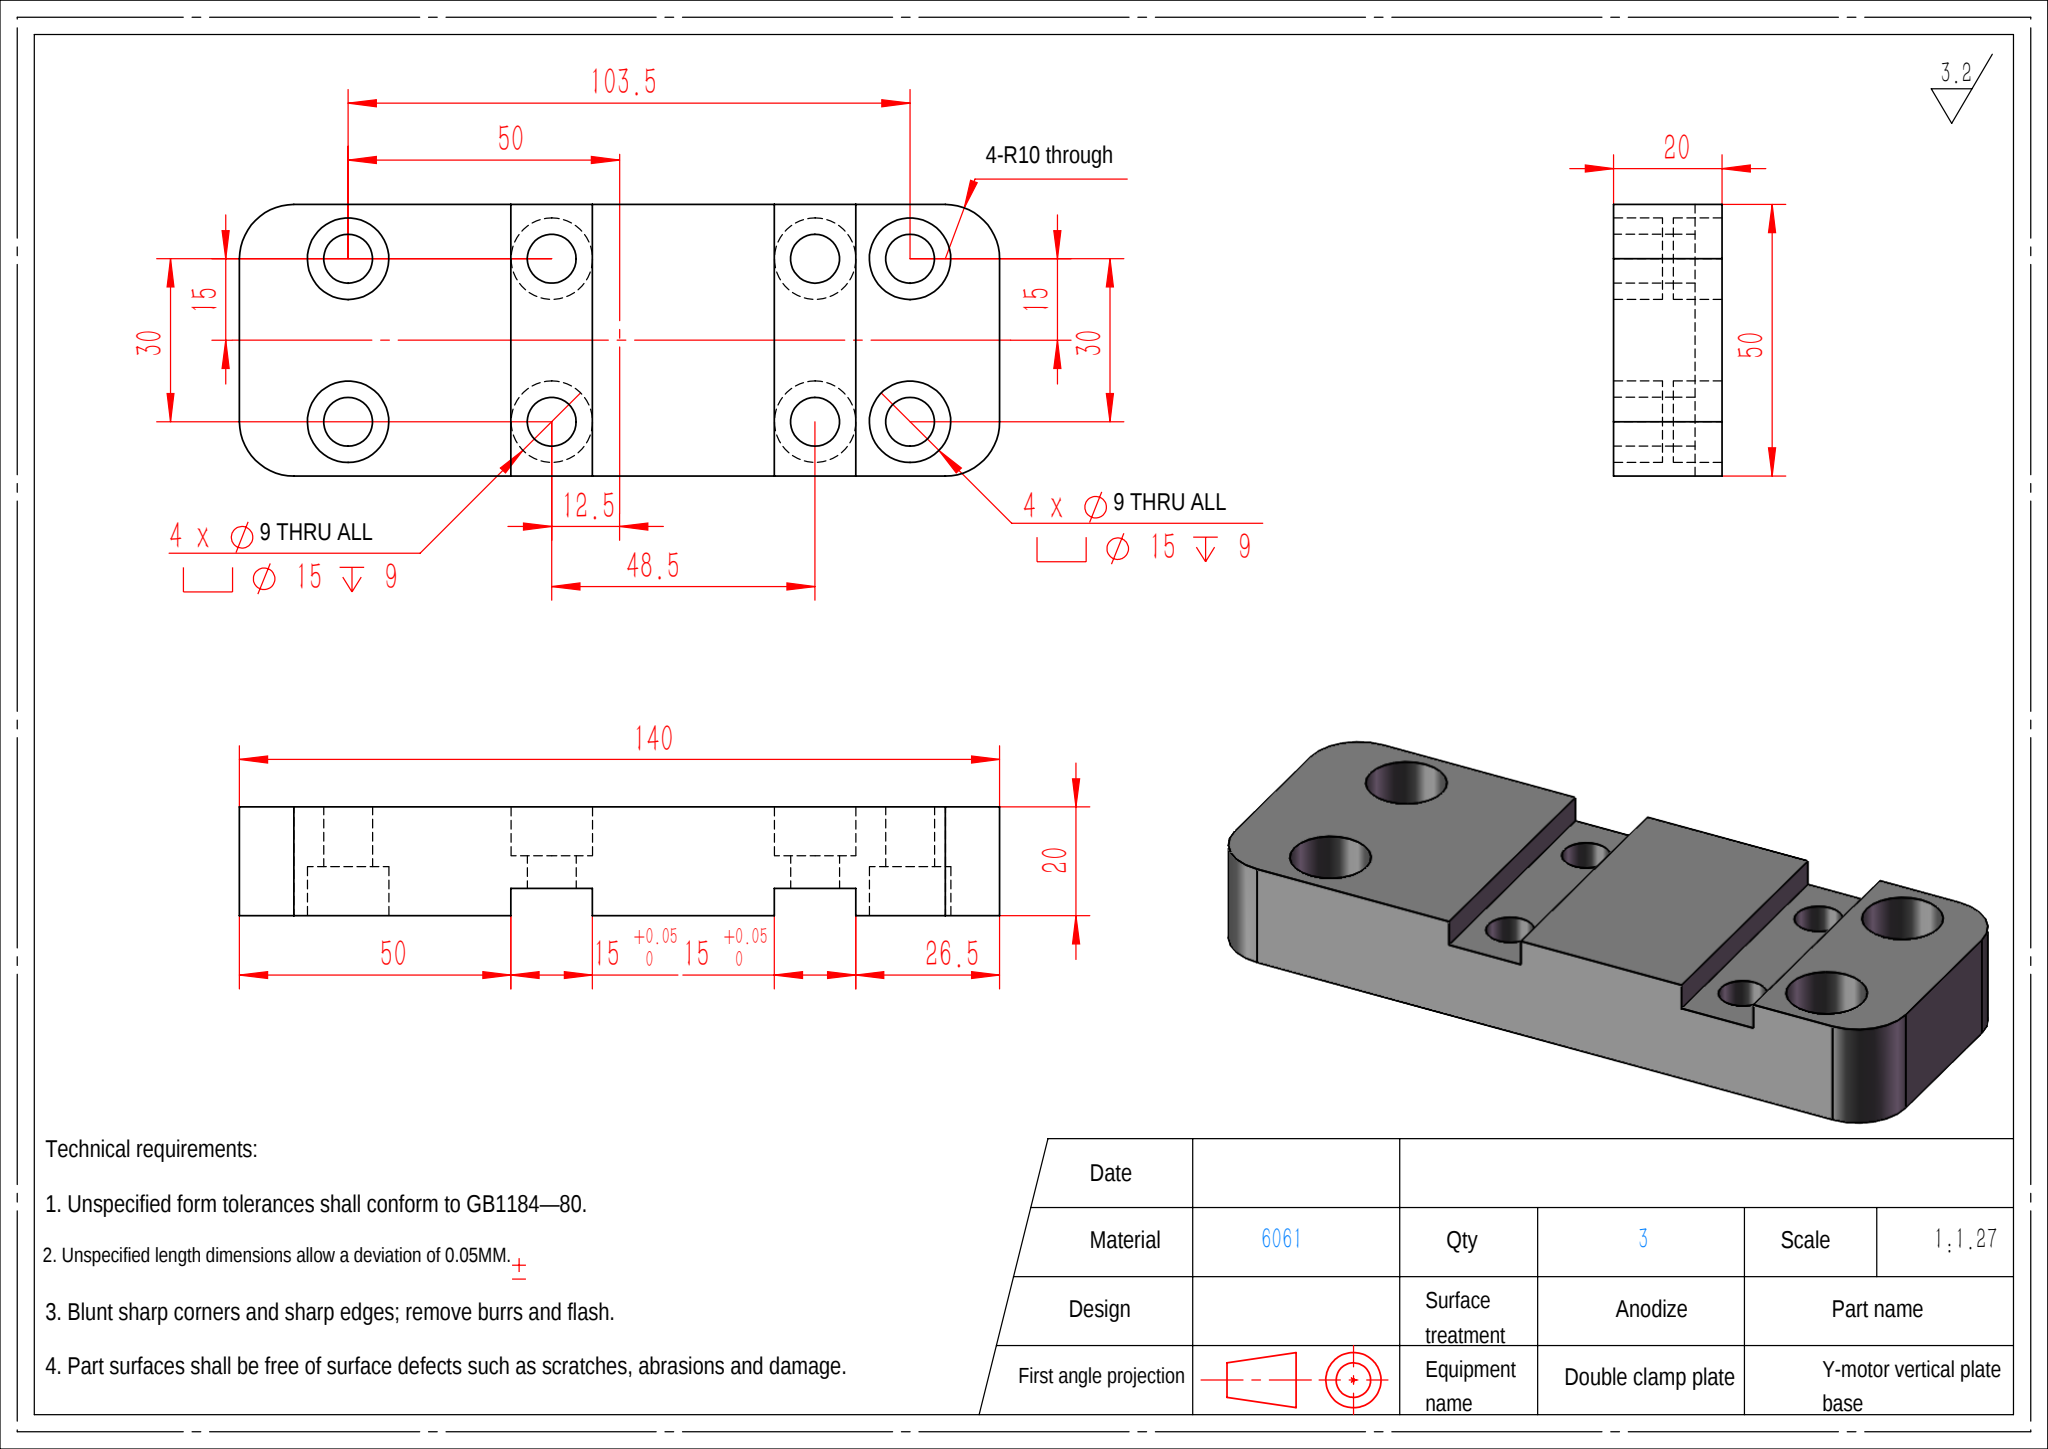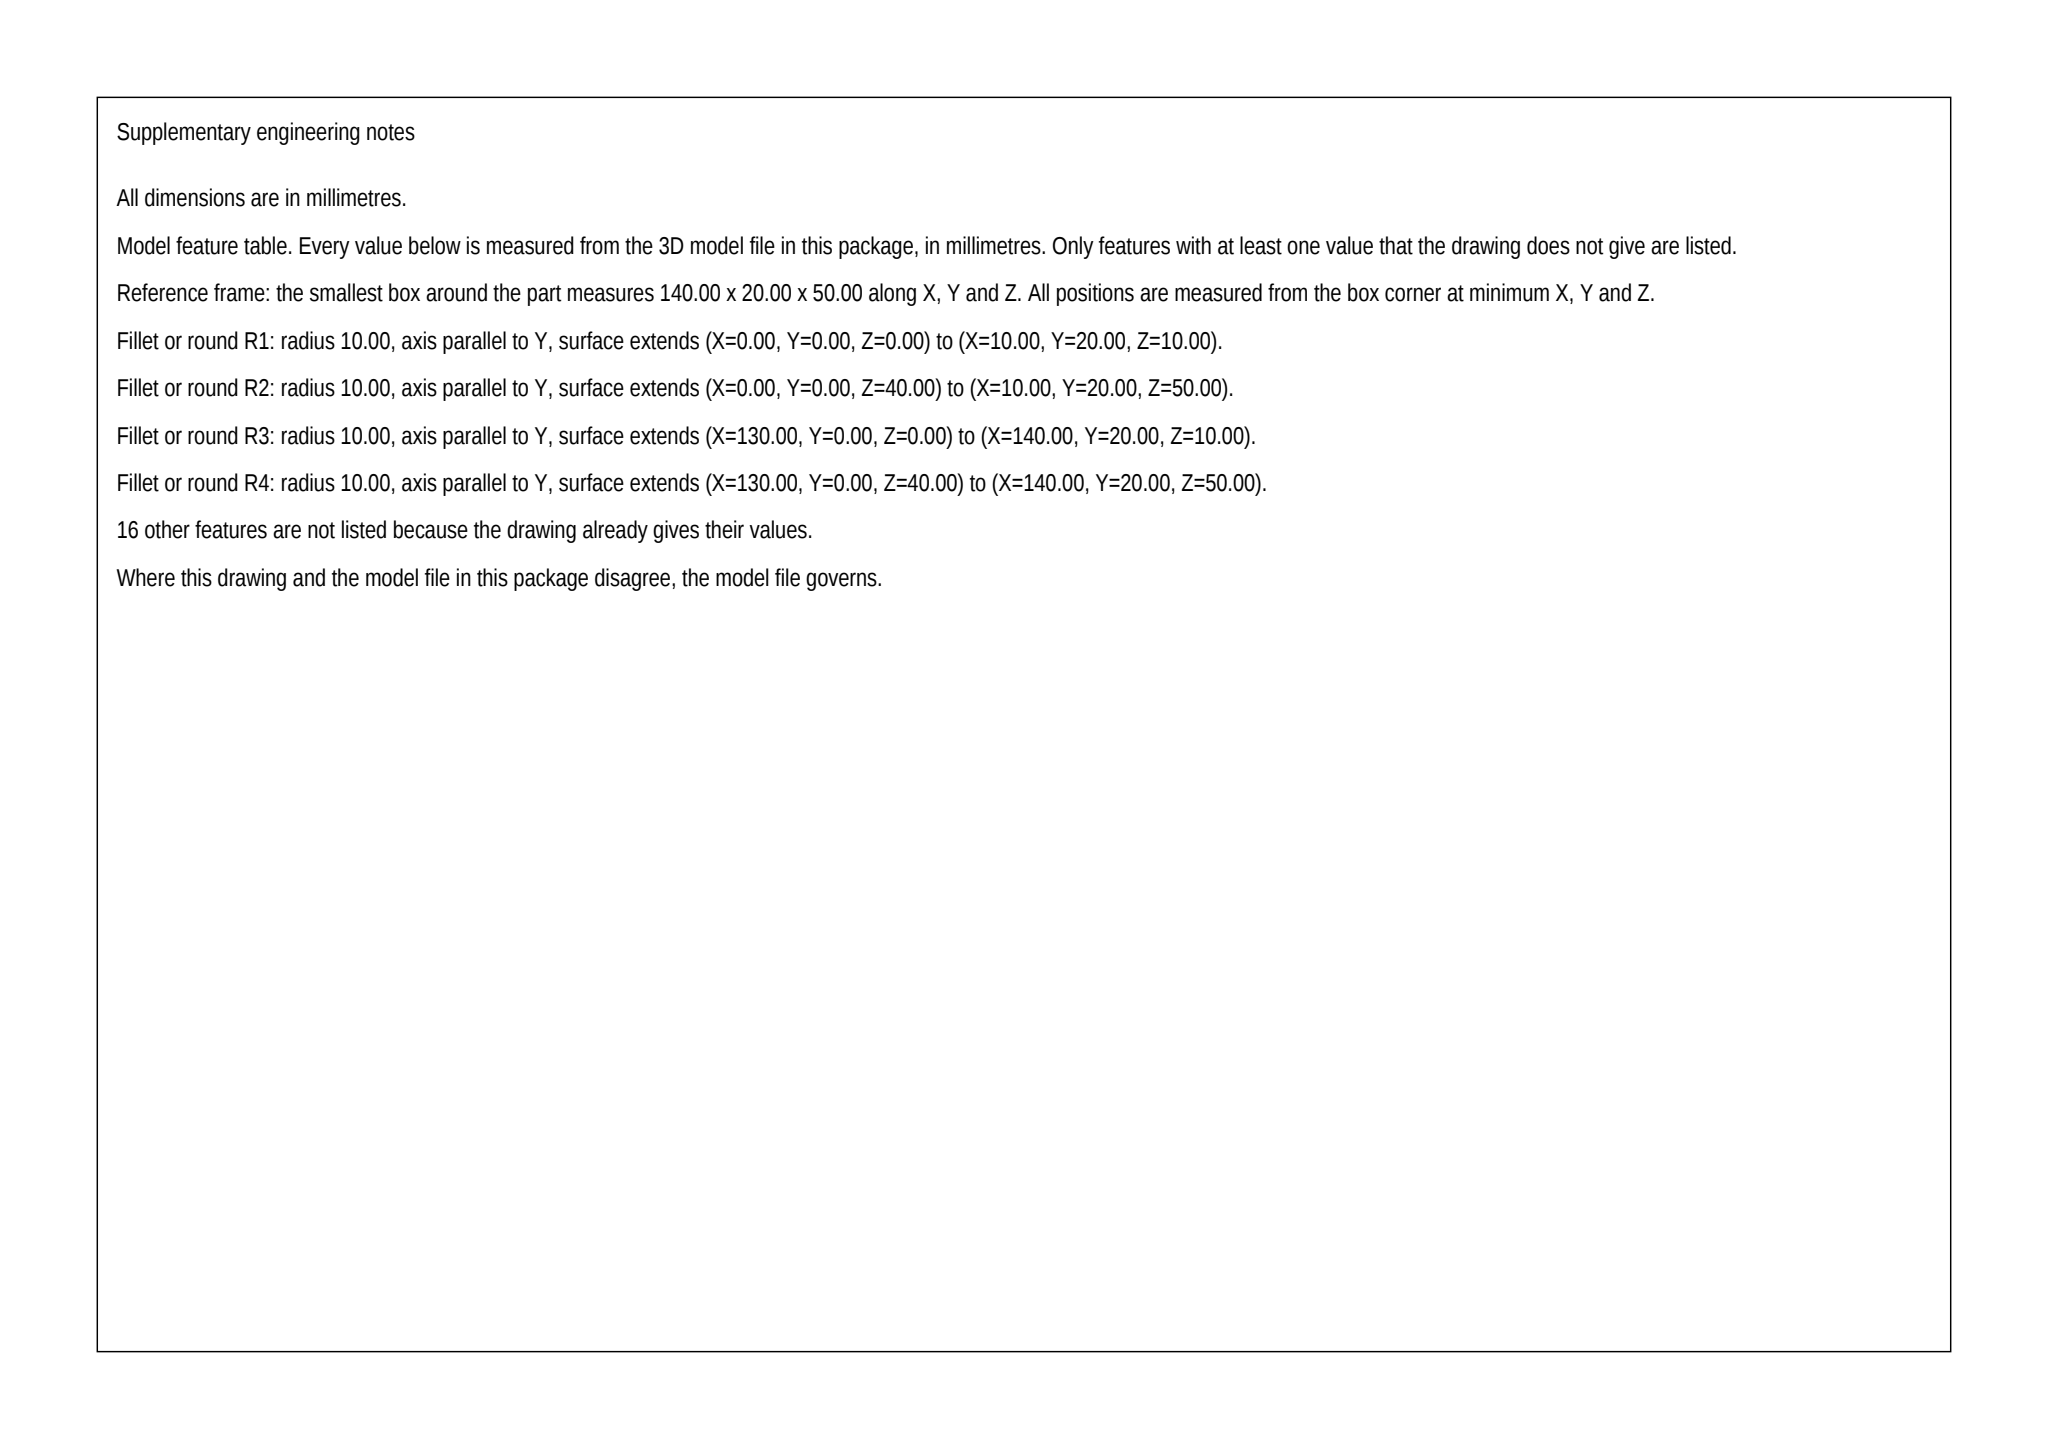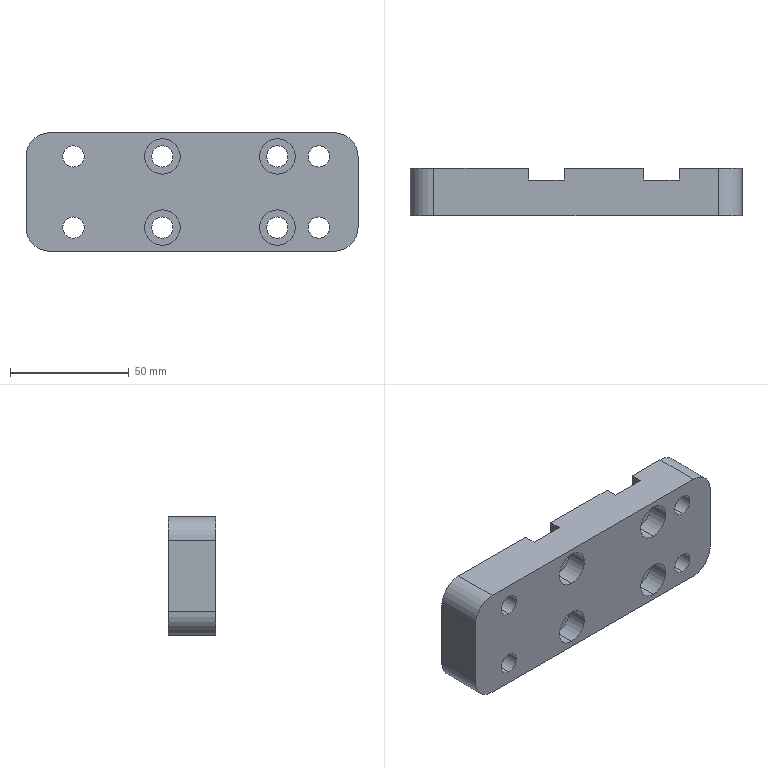Part | SolidWorks | mm | material 6061 | 1 solid | 58 faces | box 140 x 20 x 50 mm | volume 113734 mm3 | cylinder 36 | plane 22 | commonest cylinder face diameters 15 x16 9 x16 20 x4
build123d program:
from build123d import *

# Parameters (mm, degrees)
SKETCH1_W                                           = 140
SKETCH1_H                                           = 50
BOSS_EXTRUDE1_DEPTH                                 = 20
SKETCH2_W                                           = 15
SKETCH2_H                                           = 5
CUT_EXTRUDE1_DEPTH                                  = 89.318
SKETCH3_W                                           = 15
SKETCH3_H                                           = 5
CUT_EXTRUDE2_DEPTH                                  = 89.318
CYLINDRICAL_COUNTERSUNK_HOLE_FOR_M8_HEX_D           = 9
CYLINDRICAL_COUNTERSUNK_HOLE_FOR_M8_HEX_CBORE_D     = 15
CYLINDRICAL_COUNTERSUNK_HOLE_FOR_M8_HEX_CBORE_DEPTH = 9
CYLINDRICAL_COUNTERSUNK_HOLE_FOR_M8_2_D             = 9
CYLINDRICAL_COUNTERSUNK_HOLE_FOR_M8_2_DEPTH         = 20
CYLINDRICAL_COUNTERSUNK_HOLE_FOR_M8_2_CBORE_D       = 15
CYLINDRICAL_COUNTERSUNK_HOLE_FOR_M8_2_CBORE_DEPTH   = 9
FILLET1_R                                           = 10


with BuildPart() as part:
    # Sketch1 → Boss-Extrude1 (new body)
    with BuildSketch(Plane.XZ):
        Rectangle(SKETCH1_W, SKETCH1_H)
    extrude(amount=-BOSS_EXTRUDE1_DEPTH)

    # Sketch2 → Cut-Extrude1 (cut, through all)
    with BuildSketch(Plane.XY.offset(25)):
        with Locations((-12.5, 17.5)):
            Rectangle(SKETCH2_W, SKETCH2_H)
    extrude(amount=-CUT_EXTRUDE1_DEPTH, mode=Mode.SUBTRACT)

    # Sketch3 → Cut-Extrude2 (cut, through all)
    with BuildSketch(Plane.XY.offset(25)):
        with Locations((36, 17.5)):
            Rectangle(SKETCH3_W, SKETCH3_H)
    extrude(amount=-CUT_EXTRUDE2_DEPTH, mode=Mode.SUBTRACT)

    # Cylindrical Countersunk Hole for M8 Hex (through all)
    with Locations(Plane(origin=(0, 20, 0), x_dir=(1, 0, 0), z_dir=(0, 1, 0))):
        with Locations((-50, -15), (-50, 15), (53.5, 15), (53.5, -15)):
            CounterBoreHole(CYLINDRICAL_COUNTERSUNK_HOLE_FOR_M8_HEX_D / 2, CYLINDRICAL_COUNTERSUNK_HOLE_FOR_M8_HEX_CBORE_D / 2, CYLINDRICAL_COUNTERSUNK_HOLE_FOR_M8_HEX_CBORE_DEPTH)

    # Cylindrical Countersunk Hole for M8  2
    with Locations(Plane(origin=(0, 0, 0), x_dir=(-1, 0, 0), z_dir=(0, -1, 0))):
        with Locations((12.5, -15), (-36, -15), (-36, 15), (12.5, 15)):
            CounterBoreHole(CYLINDRICAL_COUNTERSUNK_HOLE_FOR_M8_2_D / 2, CYLINDRICAL_COUNTERSUNK_HOLE_FOR_M8_2_CBORE_D / 2, CYLINDRICAL_COUNTERSUNK_HOLE_FOR_M8_2_CBORE_DEPTH, depth=CYLINDRICAL_COUNTERSUNK_HOLE_FOR_M8_2_DEPTH)

    # Fillet1
    fillet1_edges = [part.edges().sort_by_distance(p)[0] for p in [
        (70, 10, 25),
        (70, 10, -25),
        (-70, 10, -25),
        (-70, 10, 25),
    ]]
    fillet(fillet1_edges, radius=FILLET1_R)


solid = part.part